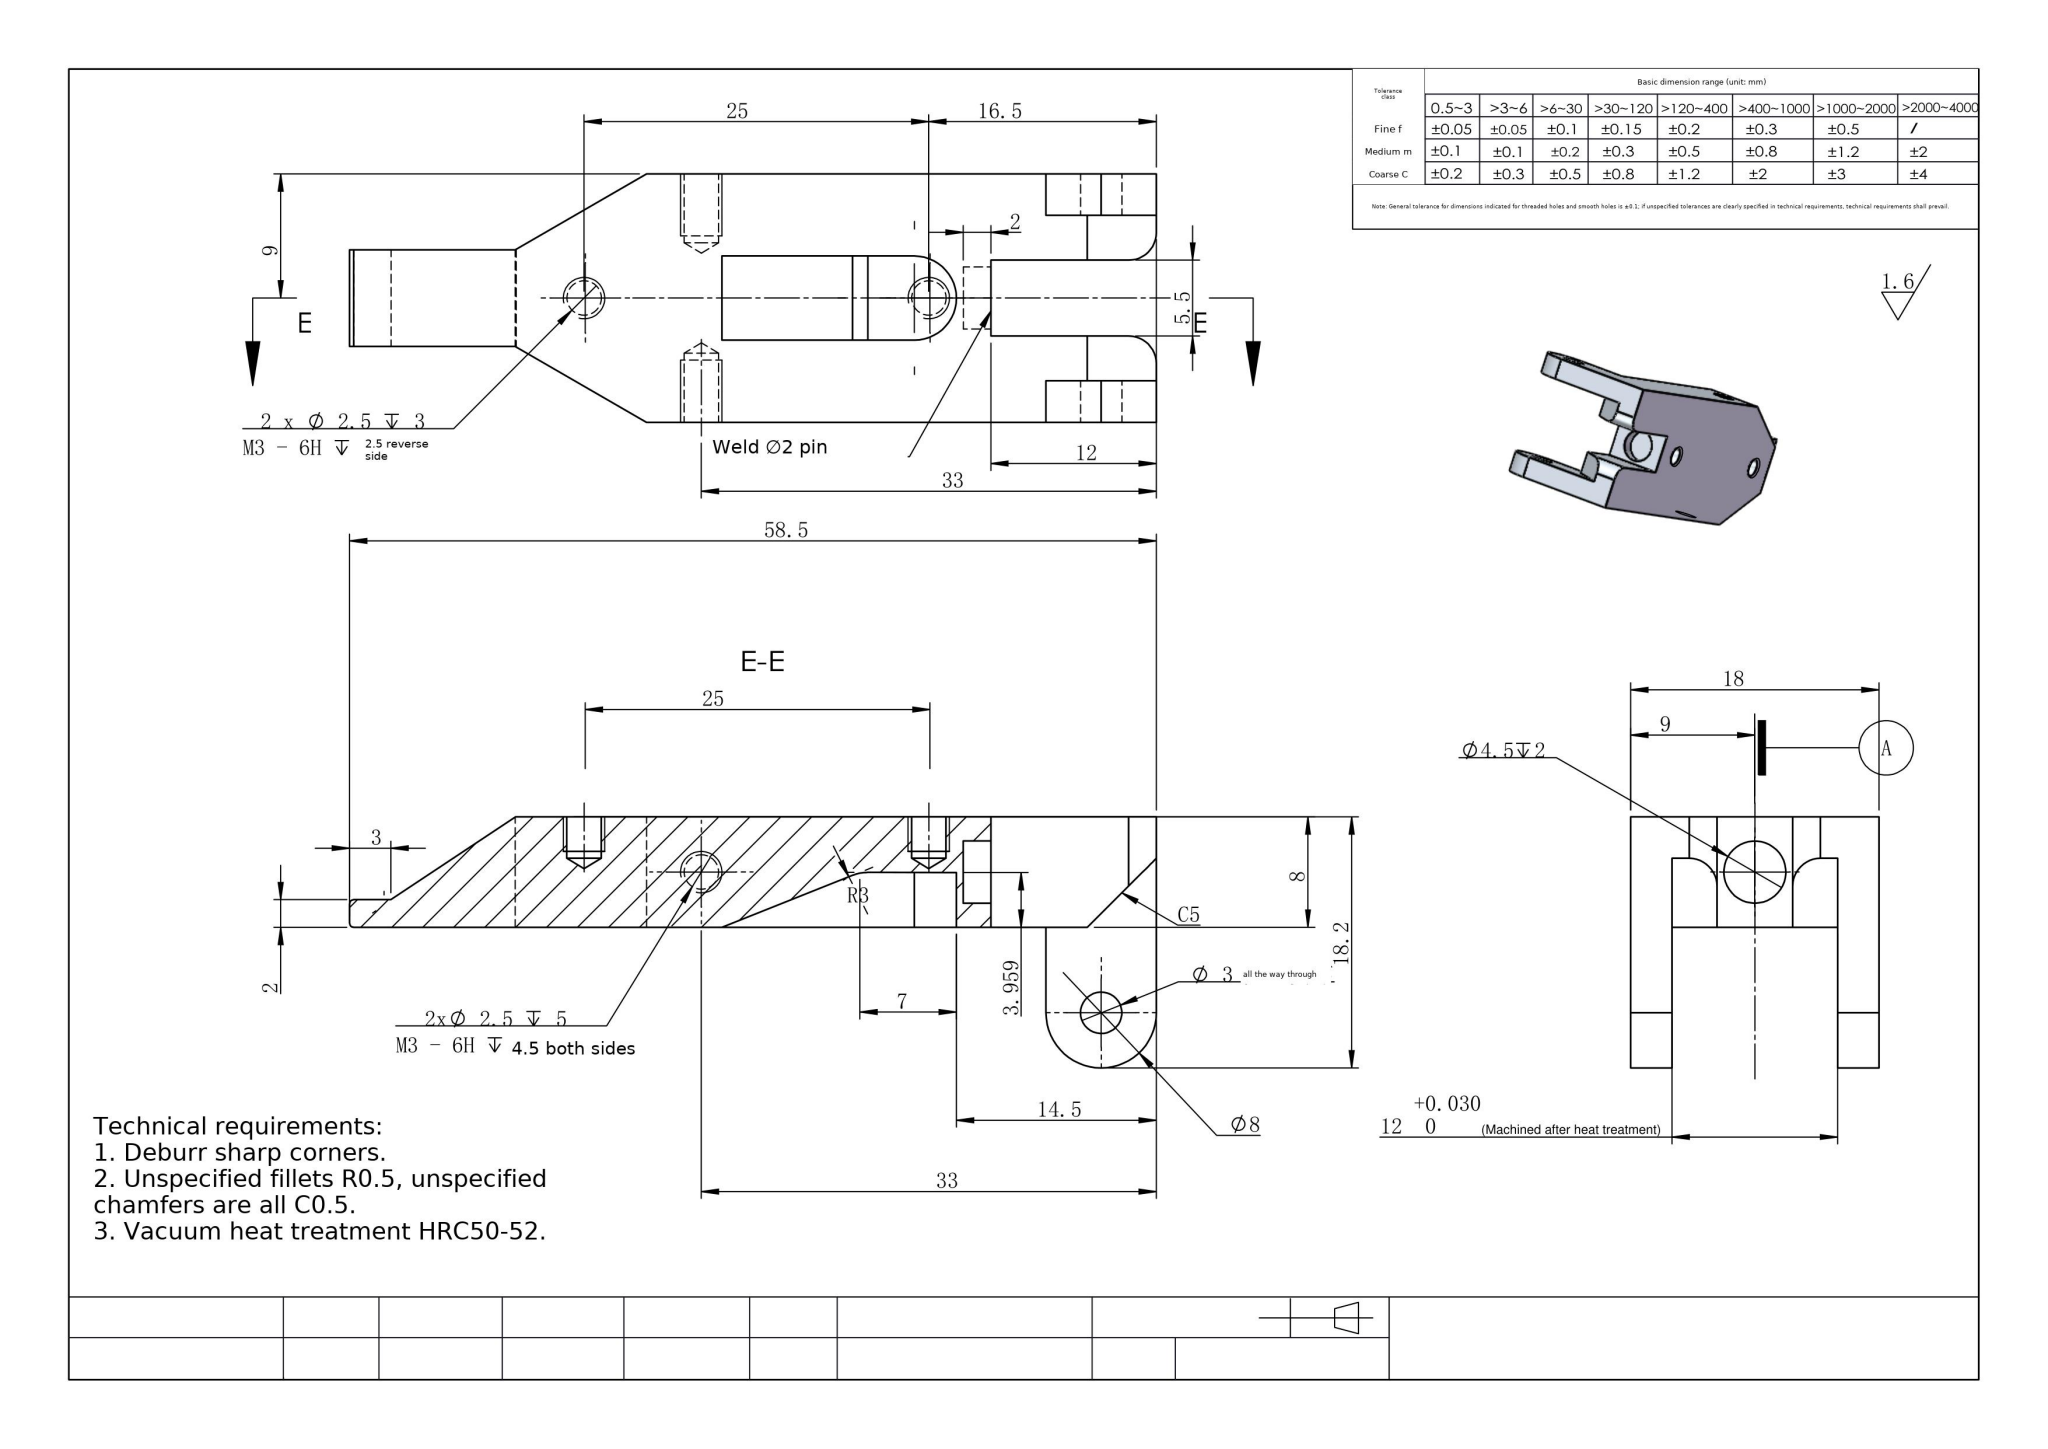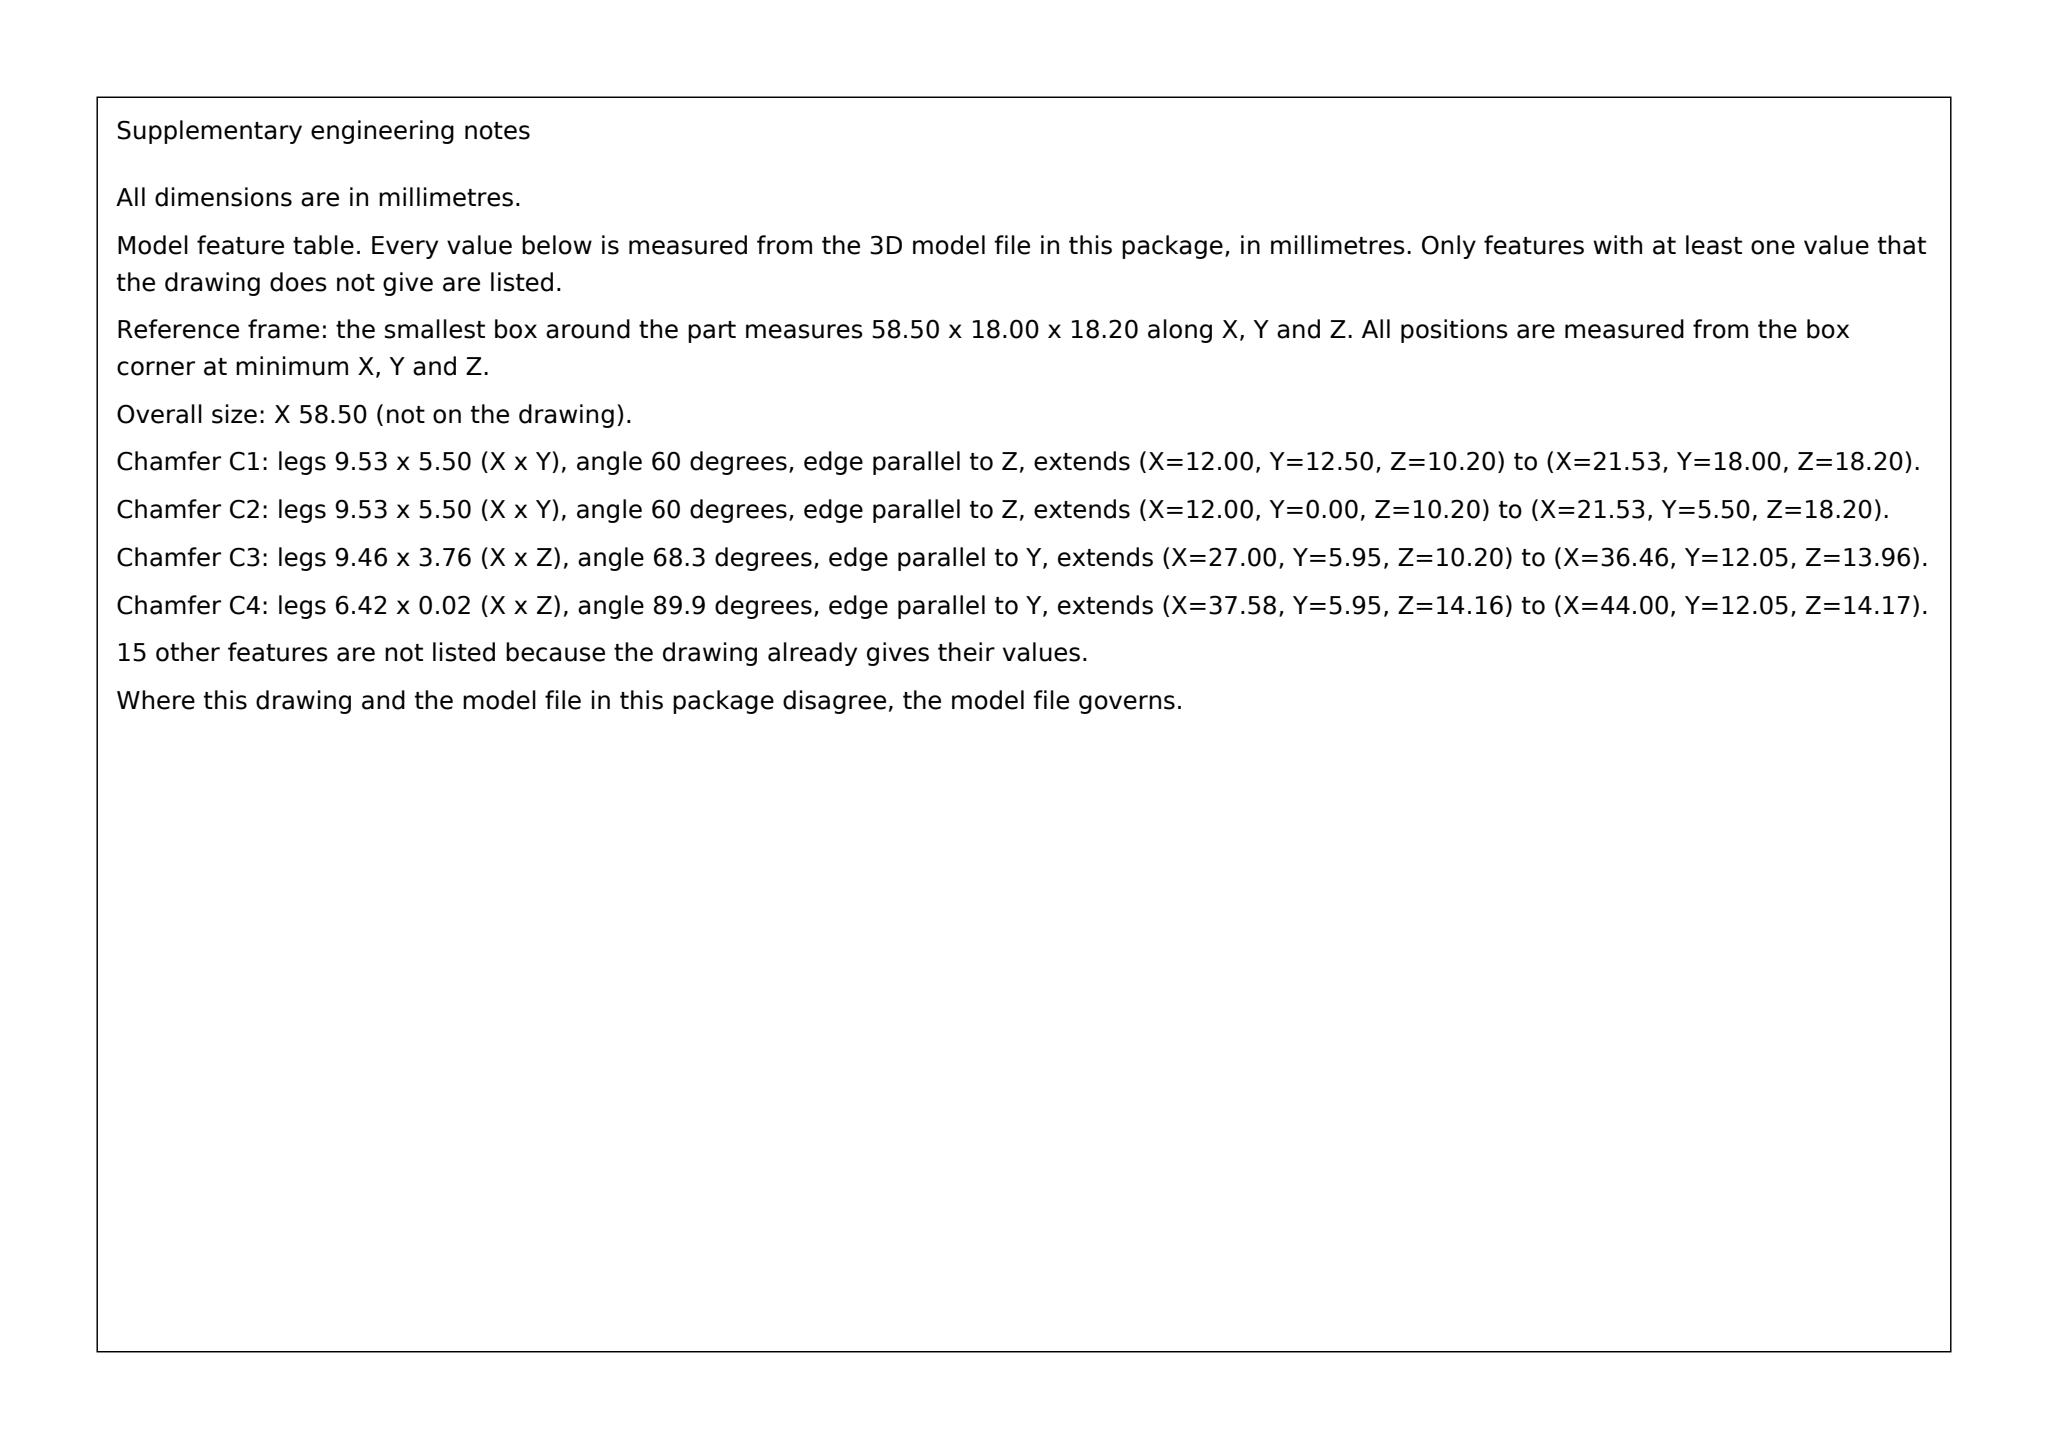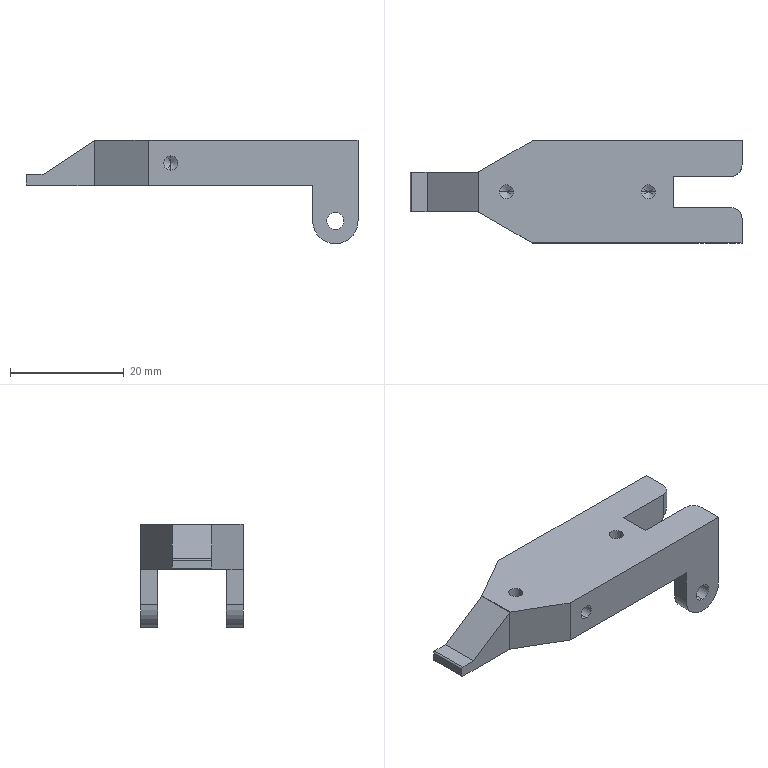Part | SolidWorks | mm | 1 solid | 62 faces | box 58.5 x 18 x 18.2 mm | volume 6034 mm3 | cylinder 27 | plane 27 | cone 8 | commonest cylinder face diameters 2.5 x8 3 x4 8 x4 0.6 x3 4.5 x2 6 x2 6.1 x2 4 x2